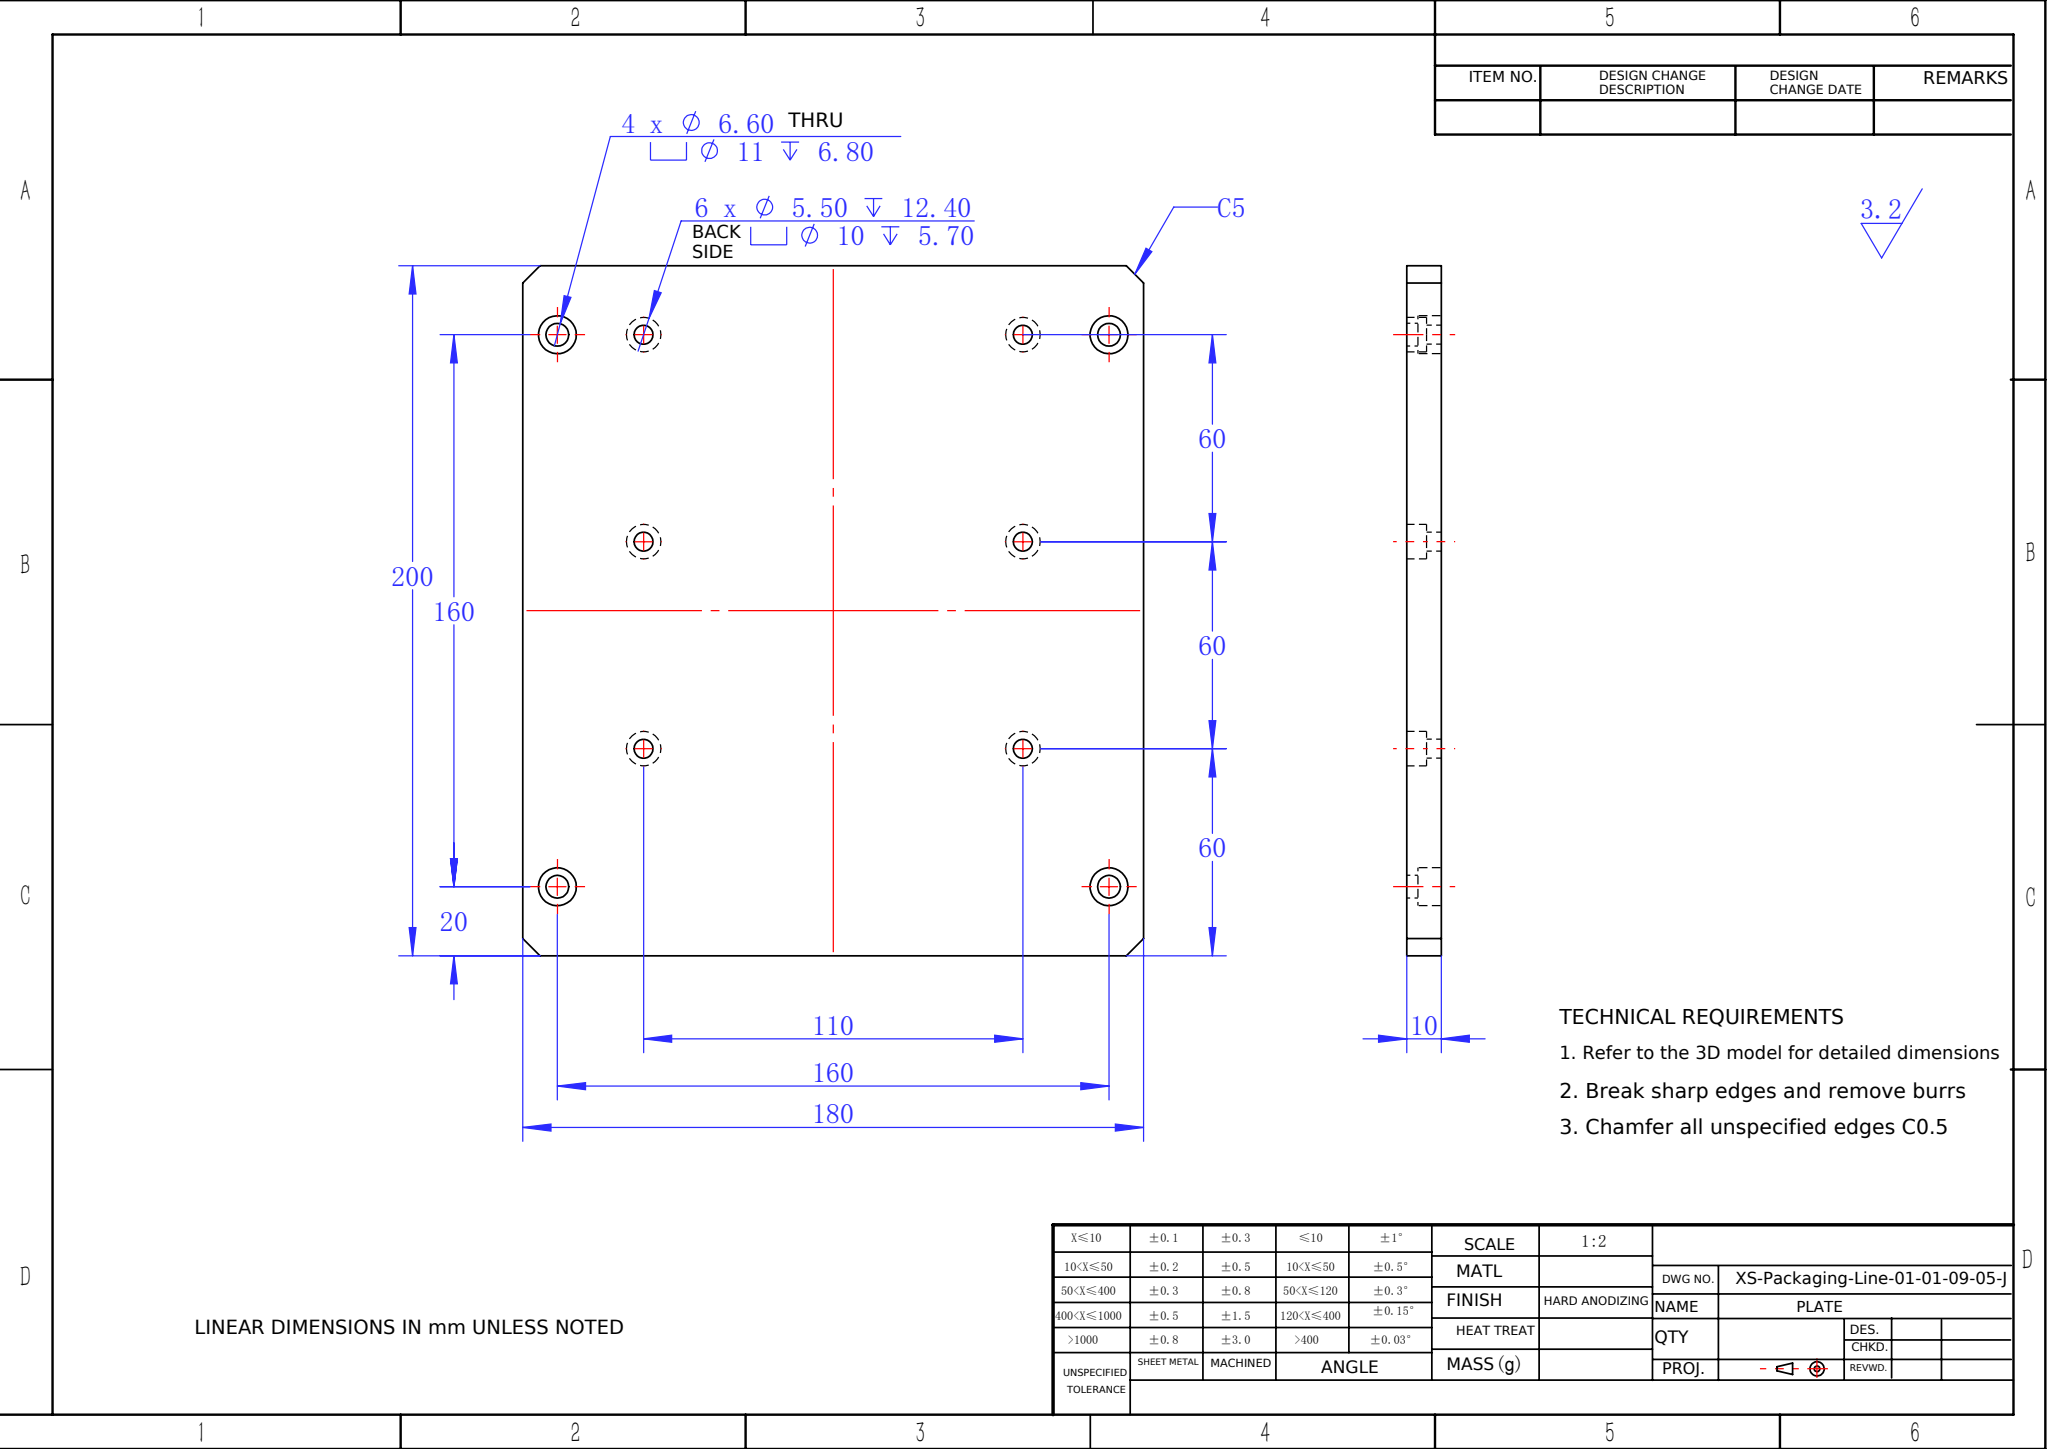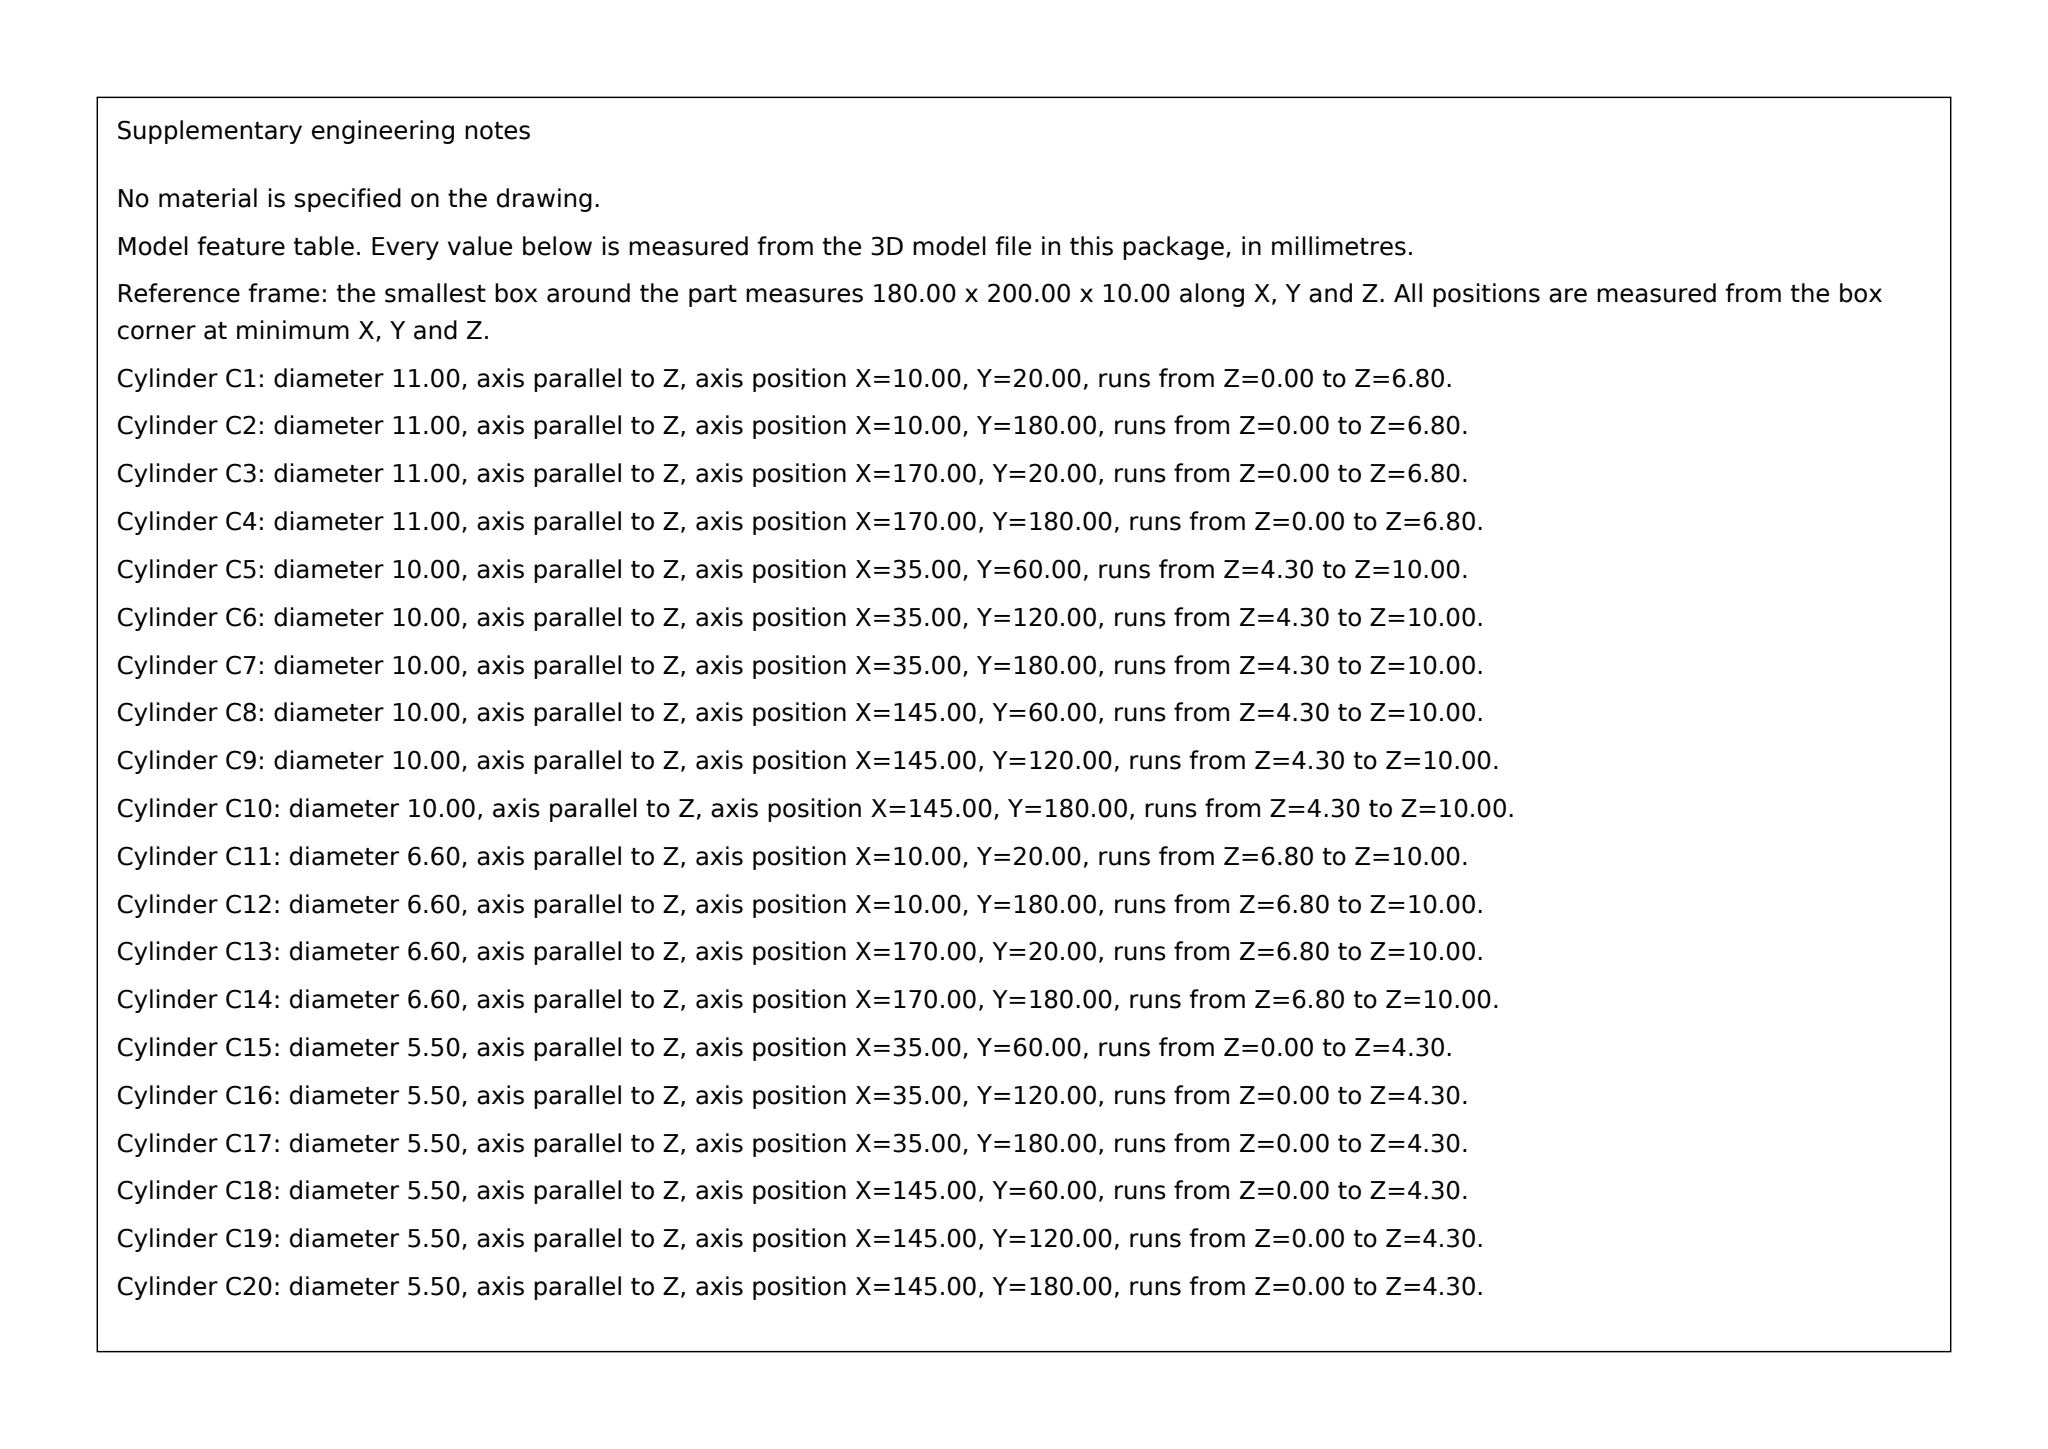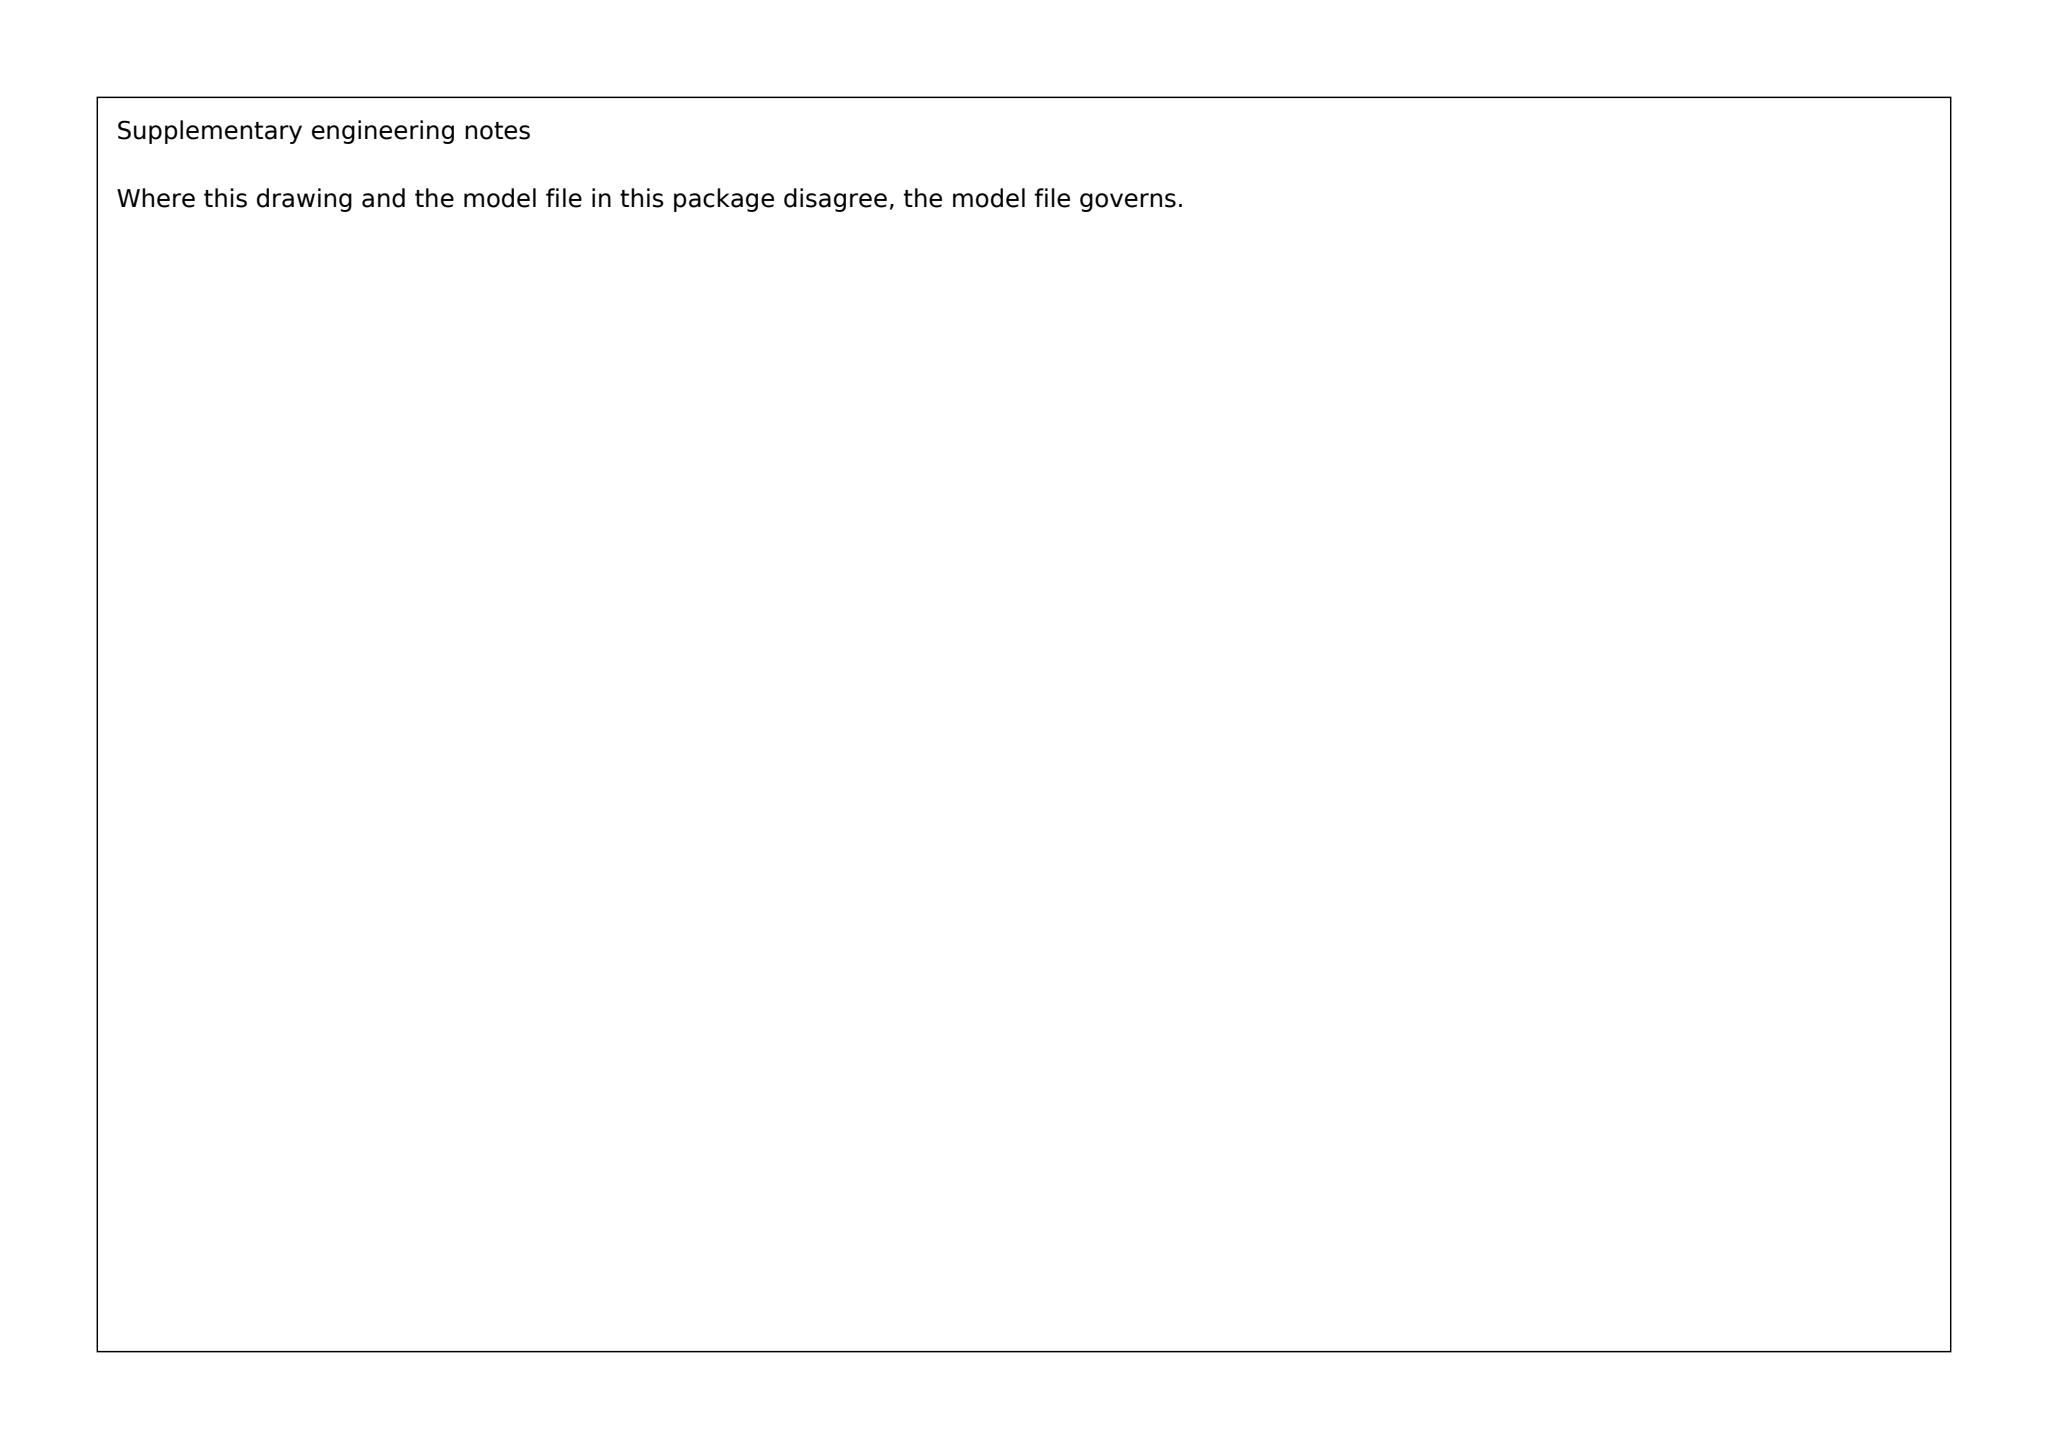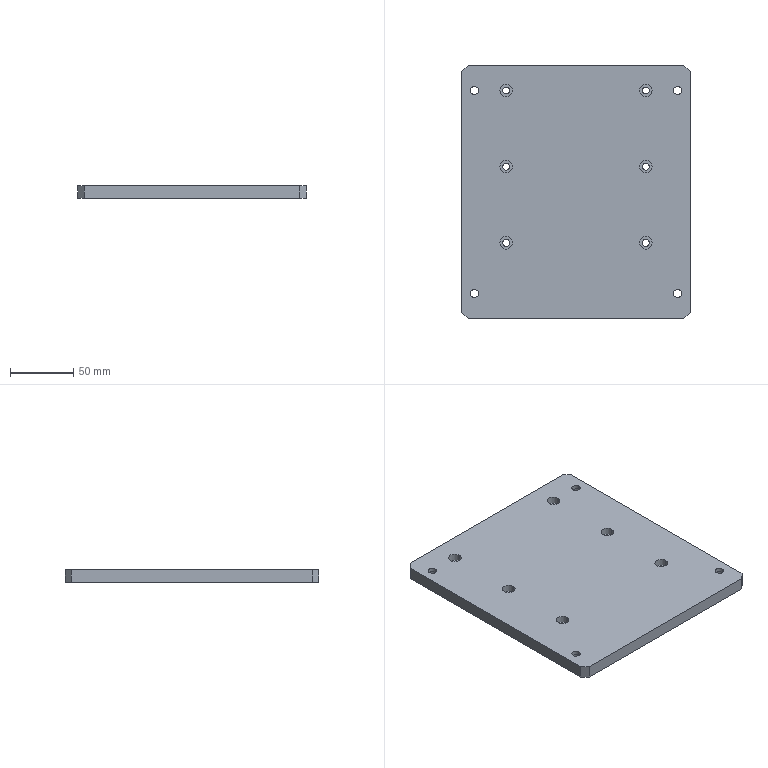Part | SolidWorks | mm | 1 solid | 60 faces | box 180 x 200 x 10 mm | volume 353178 mm3 | cylinder 40 | plane 20 | commonest cylinder face diameters 10 x12 5.5 x12 11 x8 6.6 x8
build123d program:
from build123d import *

# Parameters (mm, degrees)
SKETCH1_W                                       = 180
SKETCH1_H                                       = 200
BOSS_EXTRUDE1_DEPTH                             = 10
M6_HEX_SOCKET_HEAD_CAP_SCREW_CBORE1_D           = 6.6
M6_HEX_SOCKET_HEAD_CAP_SCREW_CBORE1_CBORE_D     = 11
M6_HEX_SOCKET_HEAD_CAP_SCREW_CBORE1_CBORE_DEPTH = 6.8
CHAMFER1_SIZE                                   = 5
M5_HEX_SOCKET_HEAD_CAP_SCREW_CBORE1_D           = 5.5
M5_HEX_SOCKET_HEAD_CAP_SCREW_CBORE1_DEPTH       = 12.4
M5_HEX_SOCKET_HEAD_CAP_SCREW_CBORE1_CBORE_D     = 10
M5_HEX_SOCKET_HEAD_CAP_SCREW_CBORE1_CBORE_DEPTH = 5.7
M5_HEX_SOCKET_HEAD_CAP_SCREW_CBORE1_TIP         = 1.652


with BuildPart() as part:
    # Sketch1 → Boss-Extrude1 (new body)
    with BuildSketch(Plane.XY):
        Rectangle(SKETCH1_W, SKETCH1_H)
    extrude(amount=BOSS_EXTRUDE1_DEPTH)

    # M6 Hex Socket Head Cap Screw CBORE1 (through all)
    with Locations(Plane(origin=(0, 0, 0), x_dir=(-1, 0, 0), z_dir=(0, 0, -1))):
        with Locations((80, 80), (-80, 80), (-80, -80), (80, -80)):
            CounterBoreHole(M6_HEX_SOCKET_HEAD_CAP_SCREW_CBORE1_D / 2, M6_HEX_SOCKET_HEAD_CAP_SCREW_CBORE1_CBORE_D / 2, M6_HEX_SOCKET_HEAD_CAP_SCREW_CBORE1_CBORE_DEPTH)

    # Chamfer1
    chamfer1_edges = [part.edges().sort_by_distance(p)[0] for p in [
        (90, -100, 5),
        (-90, -100, 5),
        (-90, 100, 5),
        (90, 100, 5),
    ]]
    chamfer(chamfer1_edges, length=CHAMFER1_SIZE)

    # M5 Hex Socket Head Cap Screw CBORE1
    with Locations(Plane.XY.offset(10)):
        with Locations((-55, 80), (-55, 20), (-55, -40), (55, 80), (55, 20), (55, -40)):
            CounterBoreHole(M5_HEX_SOCKET_HEAD_CAP_SCREW_CBORE1_D / 2, M5_HEX_SOCKET_HEAD_CAP_SCREW_CBORE1_CBORE_D / 2, M5_HEX_SOCKET_HEAD_CAP_SCREW_CBORE1_CBORE_DEPTH, depth=M5_HEX_SOCKET_HEAD_CAP_SCREW_CBORE1_DEPTH)
            with Locations((0, 0, -(M5_HEX_SOCKET_HEAD_CAP_SCREW_CBORE1_DEPTH + M5_HEX_SOCKET_HEAD_CAP_SCREW_CBORE1_TIP / 2))):  # 118° drill point
                Cone(0, M5_HEX_SOCKET_HEAD_CAP_SCREW_CBORE1_D / 2, M5_HEX_SOCKET_HEAD_CAP_SCREW_CBORE1_TIP, mode=Mode.SUBTRACT)


solid = part.part